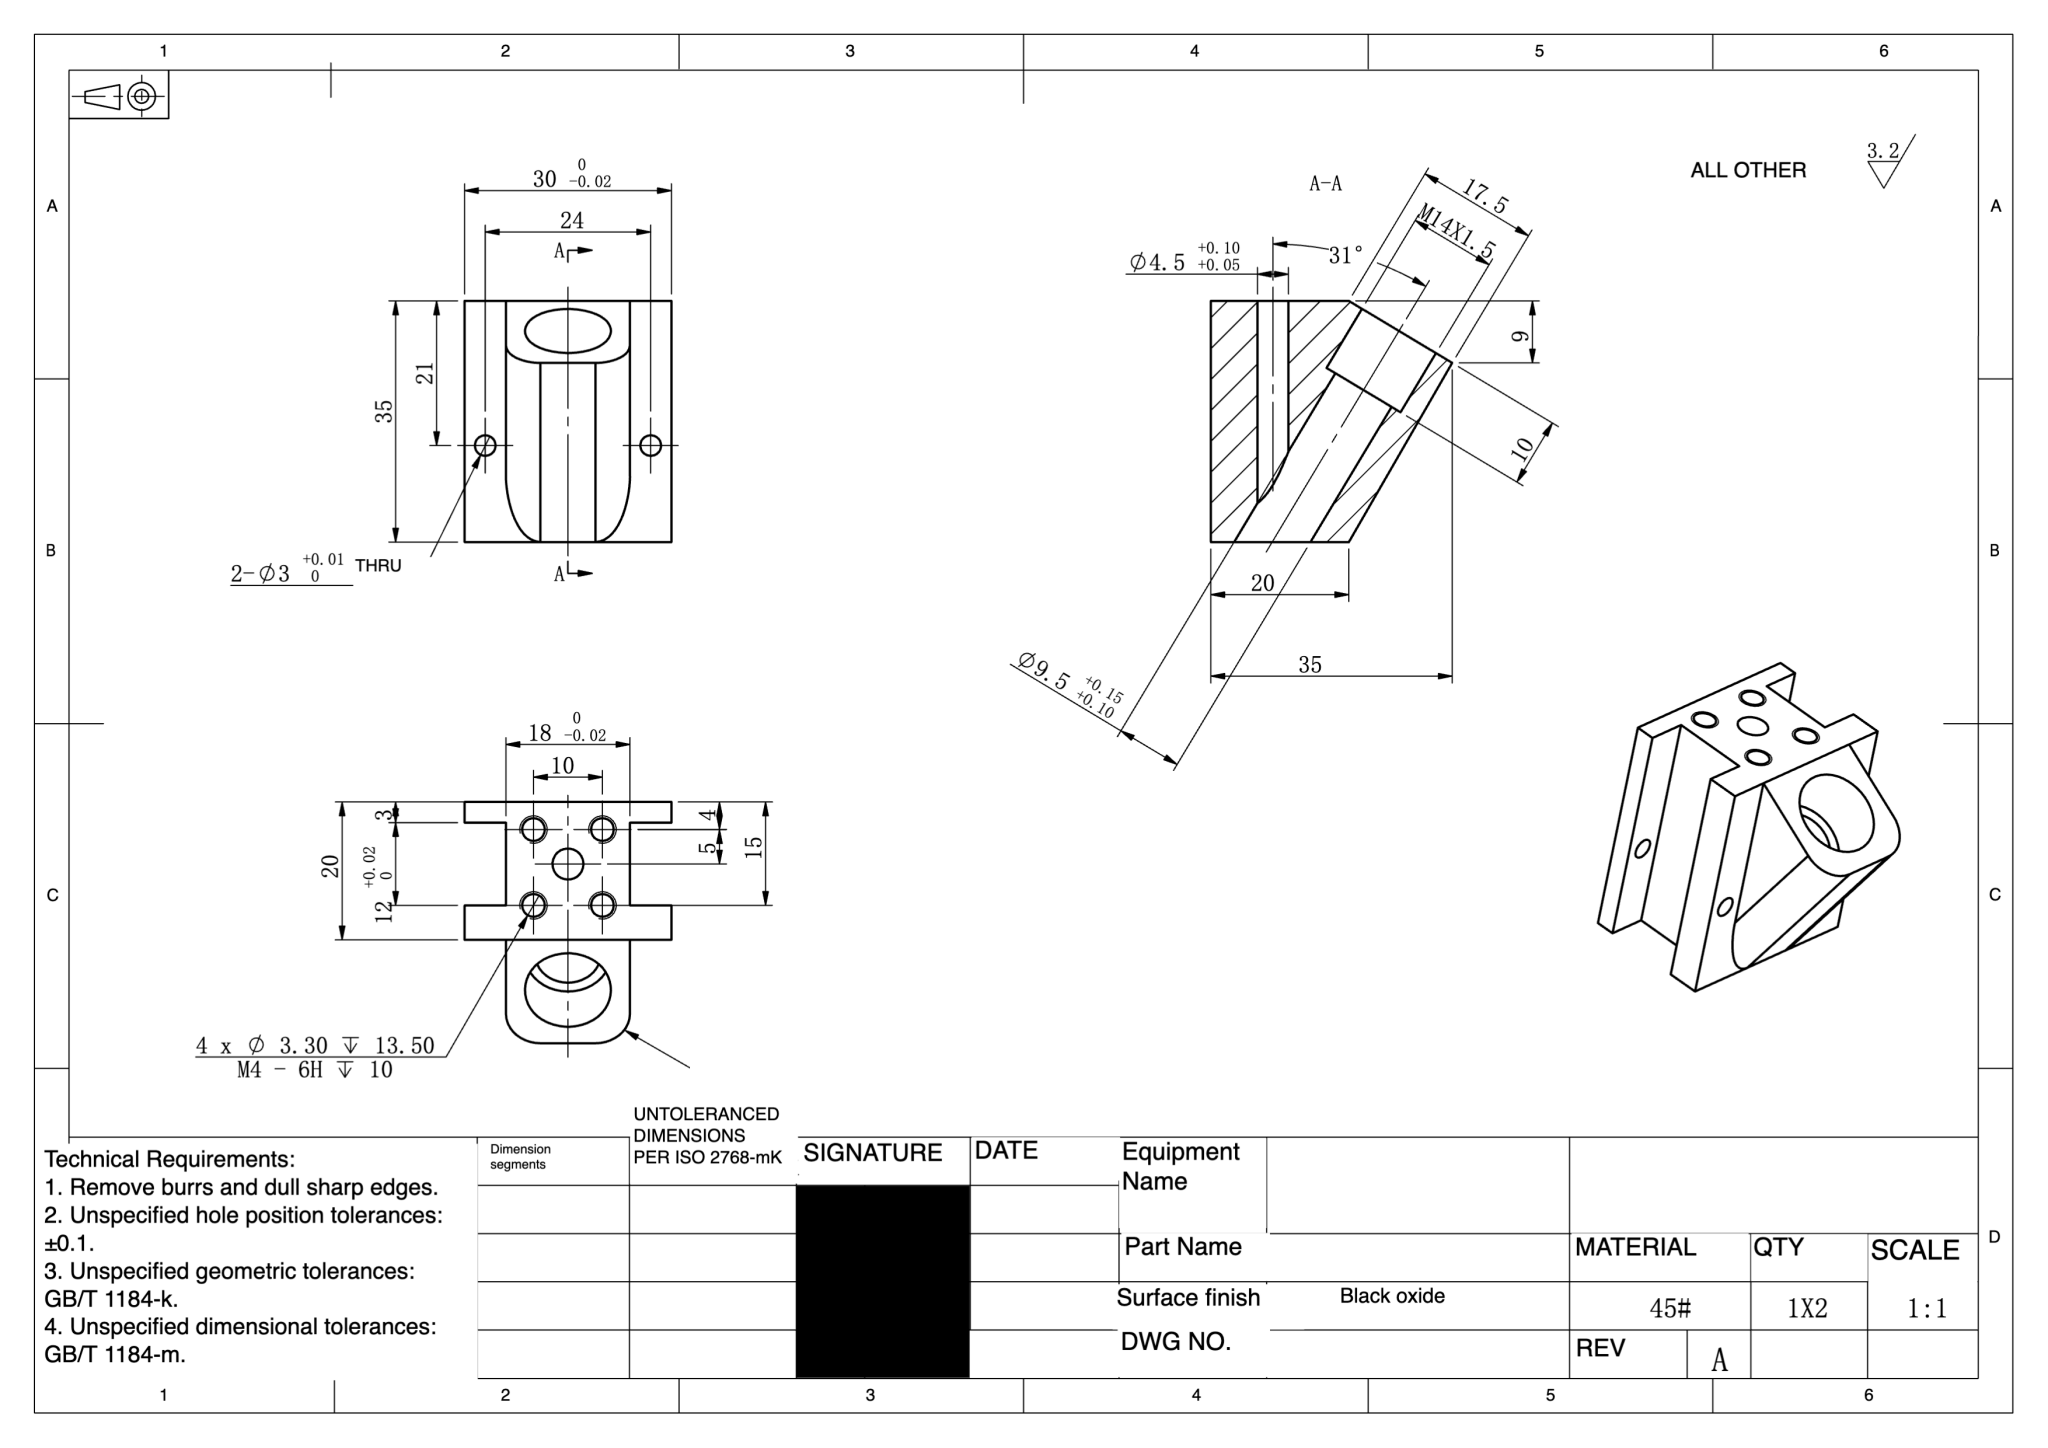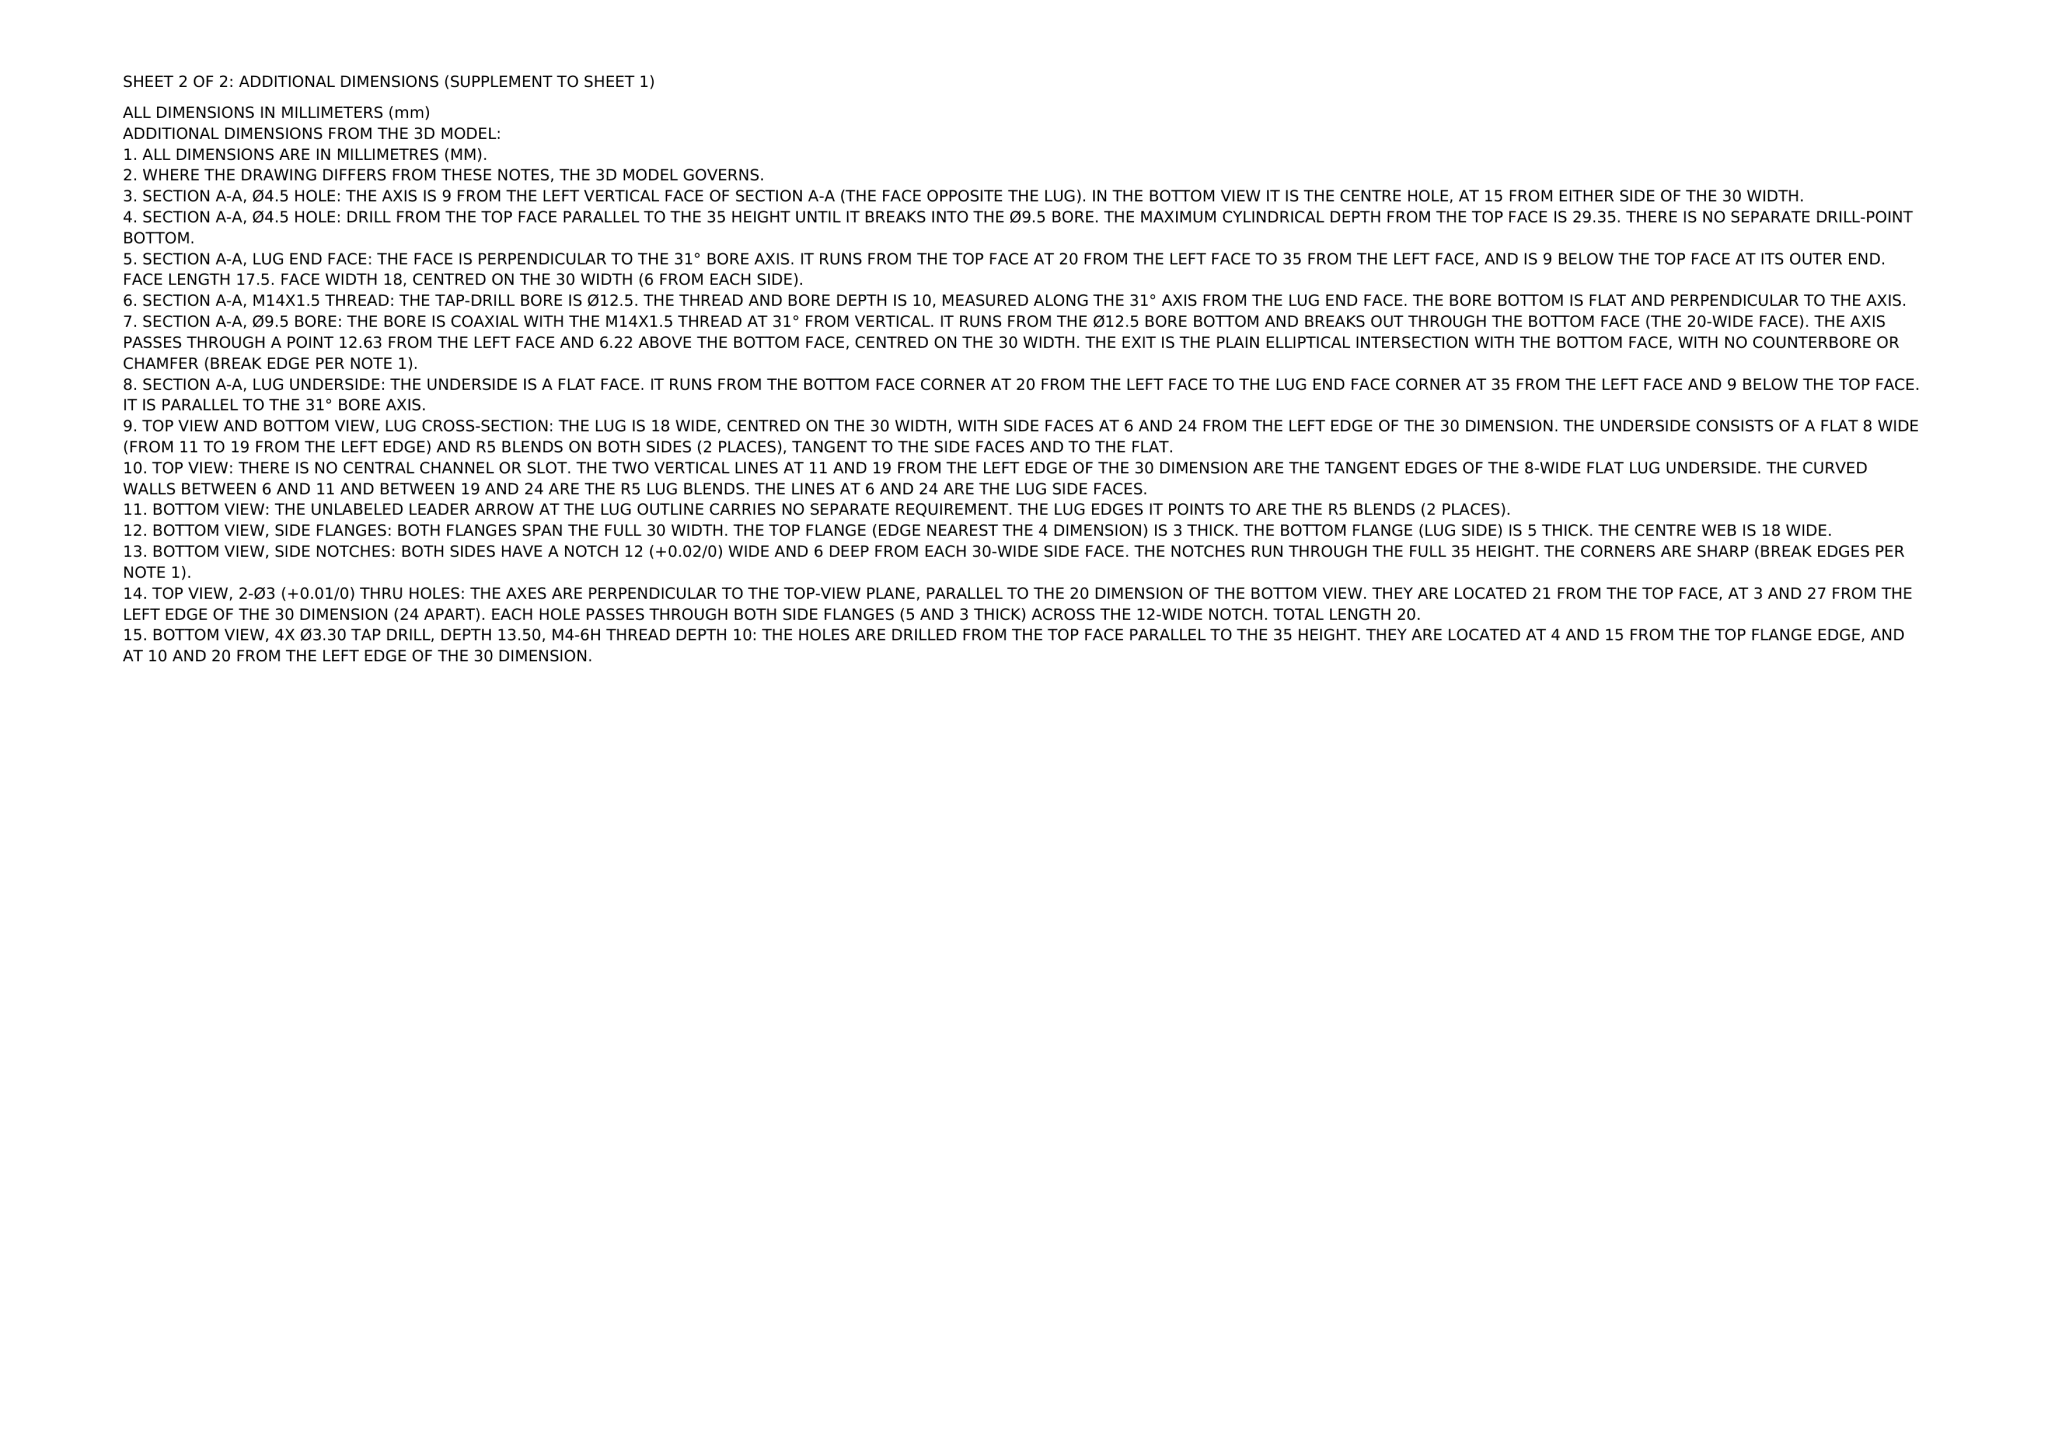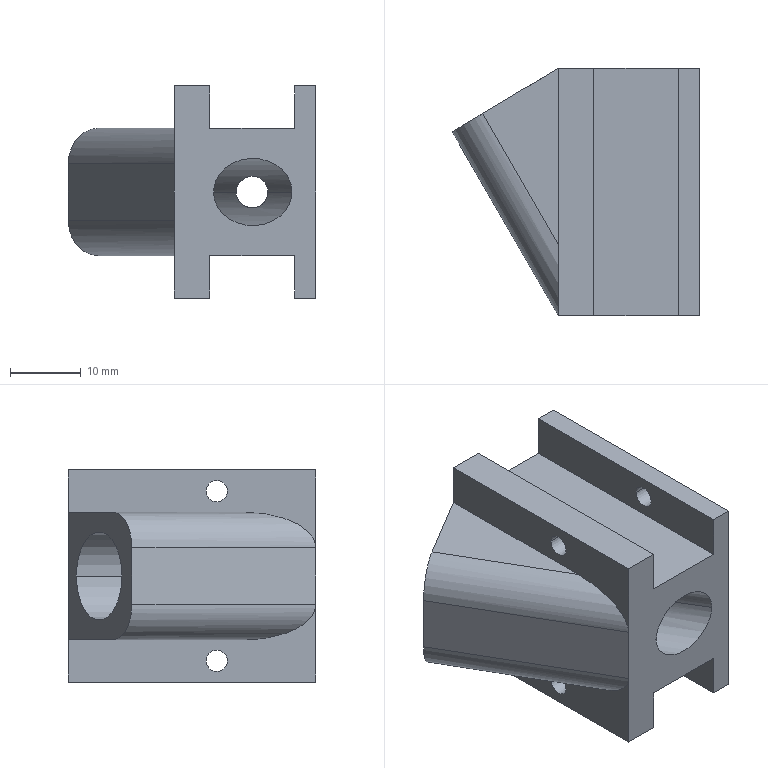Part | NX | mm | Angled Guide Block | 1 solid | 52 faces | box 35 x 35 x 30 mm | volume 16335 mm3 | cylinder 24 | plane 20 | cone 8 | commonest cylinder face diameters 3.3 x8 3 x8 12.5 x2 4.5 x2 9.5 x2 10 x2